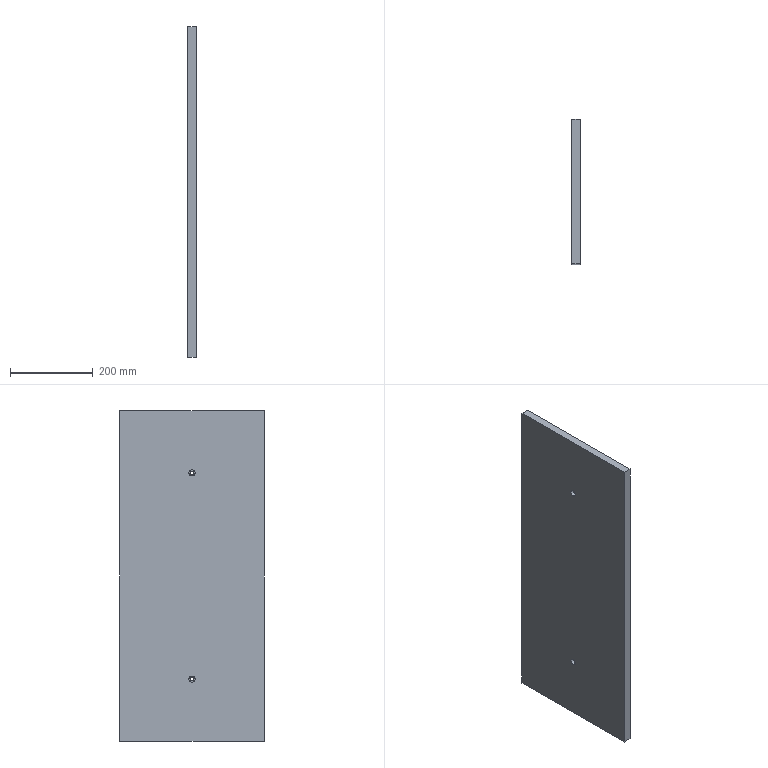Component | SolidWorks | ST60-10-1 | 1 solid | 16 faces | box 20 x 350 x 800 mm | volume 5595713 mm3 | cylinder 8 | plane 8 | commonest cylinder face diameters 15 x4 8 x4
build123d program:
from build123d import *

# Parameters (mm, degrees)
SKETCH1_W                                          = 800
SKETCH1_H                                          = 350
BOSS_EXTRUDE1_DEPTH                                = 20
HOLE_SIZE_ACCORDING_TO_TYPE_1_OF_HEXAG_D           = 8
HOLE_SIZE_ACCORDING_TO_TYPE_1_OF_HEXAG_CBORE_D     = 15
HOLE_SIZE_ACCORDING_TO_TYPE_1_OF_HEXAG_CBORE_DEPTH = 9


with BuildPart() as part:
    # Sketch1 → Boss-Extrude1 (new body)
    with BuildSketch(Plane.XY):
        with Locations((-1124.489, 541.975)):
            Rectangle(SKETCH1_W, SKETCH1_H)
    extrude(amount=BOSS_EXTRUDE1_DEPTH)

    # Hole Size _According to_ Type 1 of Hexag (through all)
    with Locations(Plane.XY.offset(20)):
        with Locations((-1374.489, 541.975), (-874.489, 541.975)):
            CounterBoreHole(HOLE_SIZE_ACCORDING_TO_TYPE_1_OF_HEXAG_D / 2, HOLE_SIZE_ACCORDING_TO_TYPE_1_OF_HEXAG_CBORE_D / 2, HOLE_SIZE_ACCORDING_TO_TYPE_1_OF_HEXAG_CBORE_DEPTH)


solid = part.part

# Placed as in the assembly
solid = solid.moved(Location((151.993, 68.479, -776.911), (0, -90, 0)))
STEP:
#1=COLOUR_RGB('',0.7922,0.8196,0.9333);
#2=FILL_AREA_STYLE_COLOUR('',#1);
#3=FILL_AREA_STYLE('',(#2));
#4=SURFACE_STYLE_FILL_AREA(#3);
#5=SURFACE_SIDE_STYLE('',(#4));
#6=SURFACE_STYLE_USAGE(.BOTH.,#5);
#7=PRESENTATION_STYLE_ASSIGNMENT((#6));
#8=CARTESIAN_POINT('',(5.551,24.034,-84.996));
#9=VERTEX_POINT('',#8);
#10=CARTESIAN_POINT('',(5.551,24.034,-84.406));
#11=VERTEX_POINT('',#10);
#12=CARTESIAN_POINT('',(5.551,24.034,-84.701));
#13=DIRECTION('',(-1.,-0.,0.));
#14=DIRECTION('',(0.,0.,1.));
#15=AXIS2_PLACEMENT_3D('',#12,#13,#14);
#16=CIRCLE('',#15,0.2953);
#17=EDGE_CURVE('',#9,#11,#16,.T.);
#18=ORIENTED_EDGE('',*,*,#17,.F.);
#19=CARTESIAN_POINT('',(5.197,24.034,-84.996));
#20=VERTEX_POINT('',#19);
#21=CARTESIAN_POINT('',(5.197,24.034,-84.996));
#22=DIRECTION('',(-1.,-0.,0.));
#23=VECTOR('',#22,39.37);
#24=LINE('',#21,#23);
#25=EDGE_CURVE('',#9,#20,#24,.T.);
#26=ORIENTED_EDGE('',*,*,#25,.T.);
#27=CARTESIAN_POINT('',(5.197,24.034,-84.406));
#28=VERTEX_POINT('',#27);
#29=CARTESIAN_POINT('',(5.197,24.034,-84.701));
#30=DIRECTION('',(-1.,-0.,0.));
#31=DIRECTION('',(0.,0.,1.));
#32=AXIS2_PLACEMENT_3D('',#29,#30,#31);
#33=CIRCLE('',#32,0.2953);
#34=EDGE_CURVE('',#20,#28,#33,.T.);
#35=ORIENTED_EDGE('',*,*,#34,.T.);
#36=CARTESIAN_POINT('',(5.197,24.034,-84.406));
#37=DIRECTION('',(-1.,-0.,0.));
#38=VECTOR('',#37,39.37);
#39=LINE('',#36,#38);
#40=EDGE_CURVE('',#11,#28,#39,.T.);
#41=ORIENTED_EDGE('',*,*,#40,.F.);
#42=EDGE_LOOP('',(#18,#26,#35,#41));
#43=FACE_OUTER_BOUND('',#42,.T.);
#44=CARTESIAN_POINT('',(5.197,24.034,-84.701));
#45=DIRECTION('',(-1.,-0.,0.));
#46=DIRECTION('',(0.,0.,1.));
#47=AXIS2_PLACEMENT_3D('',#44,#45,#46);
#48=CYLINDRICAL_SURFACE('',#47,0.2953);
#49=ADVANCED_FACE('',(#43),#48,.F.);
#50=CARTESIAN_POINT('',(5.984,24.034,-84.858));
#51=VERTEX_POINT('',#50);
#52=CARTESIAN_POINT('',(5.984,24.034,-84.543));
#53=VERTEX_POINT('',#52);
#54=CARTESIAN_POINT('',(5.984,24.034,-84.701));
#55=DIRECTION('',(-1.,-0.,0.));
#56=DIRECTION('',(0.,0.,1.));
#57=AXIS2_PLACEMENT_3D('',#54,#55,#56);
#58=CIRCLE('',#57,0.1575);
#59=EDGE_CURVE('',#51,#53,#58,.T.);
#60=ORIENTED_EDGE('',*,*,#59,.F.);
#61=CARTESIAN_POINT('',(5.551,24.034,-84.858));
#62=VERTEX_POINT('',#61);
#63=CARTESIAN_POINT('',(5.197,24.034,-84.858));
#64=DIRECTION('',(-1.,-0.,0.));
#65=VECTOR('',#64,39.37);
#66=LINE('',#63,#65);
#67=EDGE_CURVE('',#51,#62,#66,.T.);
#68=ORIENTED_EDGE('',*,*,#67,.T.);
#69=CARTESIAN_POINT('',(5.551,24.034,-84.543));
#70=VERTEX_POINT('',#69);
#71=CARTESIAN_POINT('',(5.551,24.034,-84.701));
#72=DIRECTION('',(-1.,-0.,0.));
#73=DIRECTION('',(0.,0.,1.));
#74=AXIS2_PLACEMENT_3D('',#71,#72,#73);
#75=CIRCLE('',#74,0.1575);
#76=EDGE_CURVE('',#62,#70,#75,.T.);
#77=ORIENTED_EDGE('',*,*,#76,.T.);
#78=CARTESIAN_POINT('',(5.197,24.034,-84.543));
#79=DIRECTION('',(-1.,-0.,0.));
#80=VECTOR('',#79,39.37);
#81=LINE('',#78,#80);
#82=EDGE_CURVE('',#53,#70,#81,.T.);
#83=ORIENTED_EDGE('',*,*,#82,.F.);
#84=EDGE_LOOP('',(#60,#68,#77,#83));
#85=FACE_OUTER_BOUND('',#84,.T.);
#86=CARTESIAN_POINT('',(5.197,24.034,-84.701));
#87=DIRECTION('',(-1.,-0.,0.));
#88=DIRECTION('',(0.,0.,1.));
#89=AXIS2_PLACEMENT_3D('',#86,#87,#88);
#90=CYLINDRICAL_SURFACE('',#89,0.1575);
#91=ADVANCED_FACE('',(#85),#90,.F.);
#92=CARTESIAN_POINT('',(5.551,24.034,-65.311));
#93=VERTEX_POINT('',#92);
#94=CARTESIAN_POINT('',(5.551,24.034,-64.72));
#95=VERTEX_POINT('',#94);
#96=CARTESIAN_POINT('',(5.551,24.034,-65.016));
#97=DIRECTION('',(-1.,-0.,0.));
#98=DIRECTION('',(0.,0.,1.));
#99=AXIS2_PLACEMENT_3D('',#96,#97,#98);
#100=CIRCLE('',#99,0.2953);
#101=EDGE_CURVE('',#93,#95,#100,.T.);
#102=ORIENTED_EDGE('',*,*,#101,.F.);
#103=CARTESIAN_POINT('',(5.197,24.034,-65.311));
#104=VERTEX_POINT('',#103);
#105=CARTESIAN_POINT('',(5.197,24.034,-65.311));
#106=DIRECTION('',(-1.,-0.,0.));
#107=VECTOR('',#106,39.37);
#108=LINE('',#105,#107);
#109=EDGE_CURVE('',#93,#104,#108,.T.);
#110=ORIENTED_EDGE('',*,*,#109,.T.);
#111=CARTESIAN_POINT('',(5.197,24.034,-64.72));
#112=VERTEX_POINT('',#111);
#113=CARTESIAN_POINT('',(5.197,24.034,-65.016));
#114=DIRECTION('',(-1.,-0.,0.));
#115=DIRECTION('',(0.,0.,1.));
#116=AXIS2_PLACEMENT_3D('',#113,#114,#115);
#117=CIRCLE('',#116,0.2953);
#118=EDGE_CURVE('',#104,#112,#117,.T.);
#119=ORIENTED_EDGE('',*,*,#118,.T.);
#120=CARTESIAN_POINT('',(5.197,24.034,-64.72));
#121=DIRECTION('',(-1.,-0.,0.));
#122=VECTOR('',#121,39.37);
#123=LINE('',#120,#122);
#124=EDGE_CURVE('',#95,#112,#123,.T.);
#125=ORIENTED_EDGE('',*,*,#124,.F.);
#126=EDGE_LOOP('',(#102,#110,#119,#125));
#127=FACE_OUTER_BOUND('',#126,.T.);
#128=CARTESIAN_POINT('',(5.197,24.034,-65.016));
#129=DIRECTION('',(-1.,-0.,0.));
#130=DIRECTION('',(0.,0.,1.));
#131=AXIS2_PLACEMENT_3D('',#128,#129,#130);
#132=CYLINDRICAL_SURFACE('',#131,0.2953);
#133=ADVANCED_FACE('',(#127),#132,.F.);
#134=CARTESIAN_POINT('',(5.984,24.034,-65.173));
#135=VERTEX_POINT('',#134);
#136=CARTESIAN_POINT('',(5.984,24.034,-64.858));
#137=VERTEX_POINT('',#136);
#138=CARTESIAN_POINT('',(5.984,24.034,-65.016));
#139=DIRECTION('',(-1.,-0.,0.));
#140=DIRECTION('',(0.,0.,1.));
#141=AXIS2_PLACEMENT_3D('',#138,#139,#140);
#142=CIRCLE('',#141,0.1575);
#143=EDGE_CURVE('',#135,#137,#142,.T.);
#144=ORIENTED_EDGE('',*,*,#143,.F.);
#145=CARTESIAN_POINT('',(5.551,24.034,-65.173));
#146=VERTEX_POINT('',#145);
#147=CARTESIAN_POINT('',(5.197,24.034,-65.173));
#148=DIRECTION('',(-1.,-0.,0.));
#149=VECTOR('',#148,39.37);
#150=LINE('',#147,#149);
#151=EDGE_CURVE('',#135,#146,#150,.T.);
#152=ORIENTED_EDGE('',*,*,#151,.T.);
#153=CARTESIAN_POINT('',(5.551,24.034,-64.858));
#154=VERTEX_POINT('',#153);
#155=CARTESIAN_POINT('',(5.551,24.034,-65.016));
#156=DIRECTION('',(-1.,-0.,0.));
#157=DIRECTION('',(0.,0.,1.));
#158=AXIS2_PLACEMENT_3D('',#155,#156,#157);
#159=CIRCLE('',#158,0.1575);
#160=EDGE_CURVE('',#146,#154,#159,.T.);
#161=ORIENTED_EDGE('',*,*,#160,.T.);
#162=CARTESIAN_POINT('',(5.197,24.034,-64.858));
#163=DIRECTION('',(-1.,-0.,0.));
#164=VECTOR('',#163,39.37);
#165=LINE('',#162,#164);
#166=EDGE_CURVE('',#137,#154,#165,.T.);
#167=ORIENTED_EDGE('',*,*,#166,.F.);
#168=EDGE_LOOP('',(#144,#152,#161,#167));
#169=FACE_OUTER_BOUND('',#168,.T.);
#170=CARTESIAN_POINT('',(5.197,24.034,-65.016));
#171=DIRECTION('',(-1.,-0.,0.));
#172=DIRECTION('',(0.,0.,1.));
#173=AXIS2_PLACEMENT_3D('',#170,#171,#172);
#174=CYLINDRICAL_SURFACE('',#173,0.1575);
#175=ADVANCED_FACE('',(#169),#174,.F.);
#176=CARTESIAN_POINT('',(5.984,30.923,-90.606));
#177=VERTEX_POINT('',#176);
#178=CARTESIAN_POINT('',(5.984,17.144,-90.606));
#179=VERTEX_POINT('',#178);
#180=CARTESIAN_POINT('',(5.984,30.923,-90.606));
#181=DIRECTION('',(0.,-1.,0.));
#182=VECTOR('',#181,39.37);
#183=LINE('',#180,#182);
#184=EDGE_CURVE('',#177,#179,#183,.T.);
#185=ORIENTED_EDGE('',*,*,#184,.T.);
#186=CARTESIAN_POINT('',(5.197,17.144,-90.606));
#187=VERTEX_POINT('',#186);
#188=CARTESIAN_POINT('',(5.197,17.144,-90.606));
#189=DIRECTION('',(1.,0.,-0.));
#190=VECTOR('',#189,39.37);
#191=LINE('',#188,#190);
#192=EDGE_CURVE('',#187,#179,#191,.T.);
#193=ORIENTED_EDGE('',*,*,#192,.F.);
#194=CARTESIAN_POINT('',(5.197,30.923,-90.606));
#195=VERTEX_POINT('',#194);
#196=CARTESIAN_POINT('',(5.197,30.923,-90.606));
#197=DIRECTION('',(0.,-1.,0.));
#198=VECTOR('',#197,39.37);
#199=LINE('',#196,#198);
#200=EDGE_CURVE('',#195,#187,#199,.T.);
#201=ORIENTED_EDGE('',*,*,#200,.F.);
#202=CARTESIAN_POINT('',(5.197,30.923,-90.606));
#203=DIRECTION('',(1.,0.,-0.));
#204=VECTOR('',#203,39.37);
#205=LINE('',#202,#204);
#206=EDGE_CURVE('',#195,#177,#205,.T.);
#207=ORIENTED_EDGE('',*,*,#206,.T.);
#208=EDGE_LOOP('',(#185,#193,#201,#207));
#209=FACE_OUTER_BOUND('',#208,.T.);
#210=CARTESIAN_POINT('',(5.197,30.923,-90.606));
#211=DIRECTION('',(0.,0.,1.));
#212=DIRECTION('',(-0.,1.,-0.));
#213=AXIS2_PLACEMENT_3D('',#210,#211,#212);
#214=PLANE('',#213);
#215=ADVANCED_FACE('',(#209),#214,.F.);
#216=CARTESIAN_POINT('',(5.984,17.144,-59.11));
#217=VERTEX_POINT('',#216);
#218=CARTESIAN_POINT('',(5.984,17.144,-90.606));
#219=DIRECTION('',(0.,-0.,1.));
#220=VECTOR('',#219,39.37);
#221=LINE('',#218,#220);
#222=EDGE_CURVE('',#179,#217,#221,.T.);
#223=ORIENTED_EDGE('',*,*,#222,.T.);
#224=CARTESIAN_POINT('',(5.197,17.144,-59.11));
#225=VERTEX_POINT('',#224);
#226=CARTESIAN_POINT('',(5.197,17.144,-59.11));
#227=DIRECTION('',(1.,0.,-0.));
#228=VECTOR('',#227,39.37);
#229=LINE('',#226,#228);
#230=EDGE_CURVE('',#225,#217,#229,.T.);
#231=ORIENTED_EDGE('',*,*,#230,.F.);
#232=CARTESIAN_POINT('',(5.197,17.144,-90.606));
#233=DIRECTION('',(0.,-0.,1.));
#234=VECTOR('',#233,39.37);
#235=LINE('',#232,#234);
#236=EDGE_CURVE('',#187,#225,#235,.T.);
#237=ORIENTED_EDGE('',*,*,#236,.F.);
#238=ORIENTED_EDGE('',*,*,#192,.T.);
#239=EDGE_LOOP('',(#223,#231,#237,#238));
#240=FACE_OUTER_BOUND('',#239,.T.);
#241=CARTESIAN_POINT('',(5.197,17.144,-90.606));
#242=DIRECTION('',(-0.,1.,0.));
#243=DIRECTION('',(-1.,-0.,0.));
#244=AXIS2_PLACEMENT_3D('',#241,#242,#243);
#245=PLANE('',#244);
#246=ADVANCED_FACE('',(#240),#245,.F.);
#247=CARTESIAN_POINT('',(5.984,30.923,-59.11));
#248=VERTEX_POINT('',#247);
#249=CARTESIAN_POINT('',(5.984,30.923,-59.11));
#250=DIRECTION('',(-0.,1.,0.));
#251=VECTOR('',#250,39.37);
#252=LINE('',#249,#251);
#253=EDGE_CURVE('',#217,#248,#252,.T.);
#254=ORIENTED_EDGE('',*,*,#253,.T.);
#255=CARTESIAN_POINT('',(5.197,30.923,-59.11));
#256=VERTEX_POINT('',#255);
#257=CARTESIAN_POINT('',(5.197,30.923,-59.11));
#258=DIRECTION('',(1.,0.,-0.));
#259=VECTOR('',#258,39.37);
#260=LINE('',#257,#259);
#261=EDGE_CURVE('',#256,#248,#260,.T.);
#262=ORIENTED_EDGE('',*,*,#261,.F.);
#263=CARTESIAN_POINT('',(5.197,30.923,-59.11));
#264=DIRECTION('',(-0.,1.,0.));
#265=VECTOR('',#264,39.37);
#266=LINE('',#263,#265);
#267=EDGE_CURVE('',#225,#256,#266,.T.);
#268=ORIENTED_EDGE('',*,*,#267,.F.);
#269=ORIENTED_EDGE('',*,*,#230,.T.);
#270=EDGE_LOOP('',(#254,#262,#268,#269));
#271=FACE_OUTER_BOUND('',#270,.T.);
#272=CARTESIAN_POINT('',(5.197,30.923,-59.11));
#273=DIRECTION('',(-0.,0.,-1.));
#274=DIRECTION('',(-1.,-0.,0.));
#275=AXIS2_PLACEMENT_3D('',#272,#273,#274);
#276=PLANE('',#275);
#277=ADVANCED_FACE('',(#271),#276,.F.);
#278=CARTESIAN_POINT('',(5.984,30.923,-90.606));
#279=DIRECTION('',(-0.,0.,-1.));
#280=VECTOR('',#279,39.37);
#281=LINE('',#278,#280);
#282=EDGE_CURVE('',#248,#177,#281,.T.);
#283=ORIENTED_EDGE('',*,*,#282,.T.);
#284=ORIENTED_EDGE('',*,*,#206,.F.);
#285=CARTESIAN_POINT('',(5.197,30.923,-90.606));
#286=DIRECTION('',(-0.,0.,-1.));
#287=VECTOR('',#286,39.37);
#288=LINE('',#285,#287);
#289=EDGE_CURVE('',#256,#195,#288,.T.);
#290=ORIENTED_EDGE('',*,*,#289,.F.);
#291=ORIENTED_EDGE('',*,*,#261,.T.);
#292=EDGE_LOOP('',(#283,#284,#290,#291));
#293=FACE_OUTER_BOUND('',#292,.T.);
#294=CARTESIAN_POINT('',(5.197,30.923,-90.606));
#295=DIRECTION('',(0.,-1.,-0.));
#296=DIRECTION('',(1.,0.,-0.));
#297=AXIS2_PLACEMENT_3D('',#294,#295,#296);
#298=PLANE('',#297);
#299=ADVANCED_FACE('',(#293),#298,.F.);
#300=CARTESIAN_POINT('',(5.197,24.034,-84.701));
#301=DIRECTION('',(-1.,-0.,0.));
#302=DIRECTION('',(0.,0.,1.));
#303=AXIS2_PLACEMENT_3D('',#300,#301,#302);
#304=CIRCLE('',#303,0.2953);
#305=EDGE_CURVE('',#28,#20,#304,.T.);
#306=ORIENTED_EDGE('',*,*,#305,.F.);
#307=ORIENTED_EDGE('',*,*,#34,.F.);
#308=EDGE_LOOP('',(#306,#307));
#309=FACE_BOUND('',#308,.T.);
#310=CARTESIAN_POINT('',(5.197,24.034,-65.016));
#311=DIRECTION('',(-1.,-0.,0.));
#312=DIRECTION('',(0.,0.,1.));
#313=AXIS2_PLACEMENT_3D('',#310,#311,#312);
#314=CIRCLE('',#313,0.2953);
#315=EDGE_CURVE('',#112,#104,#314,.T.);
#316=ORIENTED_EDGE('',*,*,#315,.F.);
#317=ORIENTED_EDGE('',*,*,#118,.F.);
#318=EDGE_LOOP('',(#316,#317));
#319=FACE_BOUND('',#318,.T.);
#320=ORIENTED_EDGE('',*,*,#200,.T.);
#321=ORIENTED_EDGE('',*,*,#236,.T.);
#322=ORIENTED_EDGE('',*,*,#267,.T.);
#323=ORIENTED_EDGE('',*,*,#289,.T.);
#324=EDGE_LOOP('',(#320,#321,#322,#323));
#325=FACE_OUTER_BOUND('',#324,.T.);
#326=CARTESIAN_POINT('',(5.197,2.696,-30.587));
#327=DIRECTION('',(-1.,-0.,0.));
#328=DIRECTION('',(0.,-0.,1.));
#329=AXIS2_PLACEMENT_3D('',#326,#327,#328);
#330=PLANE('',#329);
#331=ADVANCED_FACE('',(#309,#319,#325),#330,.T.);
#332=CARTESIAN_POINT('',(5.984,24.034,-84.701));
#333=DIRECTION('',(-1.,-0.,0.));
#334=DIRECTION('',(0.,0.,1.));
#335=AXIS2_PLACEMENT_3D('',#332,#333,#334);
#336=CIRCLE('',#335,0.1575);
#337=EDGE_CURVE('',#53,#51,#336,.T.);
#338=ORIENTED_EDGE('',*,*,#337,.T.);
#339=ORIENTED_EDGE('',*,*,#59,.T.);
#340=EDGE_LOOP('',(#338,#339));
#341=FACE_BOUND('',#340,.T.);
#342=CARTESIAN_POINT('',(5.984,24.034,-65.016));
#343=DIRECTION('',(-1.,-0.,0.));
#344=DIRECTION('',(0.,0.,1.));
#345=AXIS2_PLACEMENT_3D('',#342,#343,#344);
#346=CIRCLE('',#345,0.1575);
#347=EDGE_CURVE('',#137,#135,#346,.T.);
#348=ORIENTED_EDGE('',*,*,#347,.T.);
#349=ORIENTED_EDGE('',*,*,#143,.T.);
#350=EDGE_LOOP('',(#348,#349));
#351=FACE_BOUND('',#350,.T.);
#352=ORIENTED_EDGE('',*,*,#184,.F.);
#353=ORIENTED_EDGE('',*,*,#282,.F.);
#354=ORIENTED_EDGE('',*,*,#253,.F.);
#355=ORIENTED_EDGE('',*,*,#222,.F.);
#356=EDGE_LOOP('',(#352,#353,#354,#355));
#357=FACE_OUTER_BOUND('',#356,.T.);
#358=CARTESIAN_POINT('',(5.984,2.696,-30.587));
#359=DIRECTION('',(-1.,-0.,0.));
#360=DIRECTION('',(0.,-0.,1.));
#361=AXIS2_PLACEMENT_3D('',#358,#359,#360);
#362=PLANE('',#361);
#363=ADVANCED_FACE('',(#341,#351,#357),#362,.F.);
#364=ORIENTED_EDGE('',*,*,#151,.F.);
#365=ORIENTED_EDGE('',*,*,#347,.F.);
#366=ORIENTED_EDGE('',*,*,#166,.T.);
#367=CARTESIAN_POINT('',(5.551,24.034,-65.016));
#368=DIRECTION('',(-1.,-0.,0.));
#369=DIRECTION('',(0.,0.,1.));
#370=AXIS2_PLACEMENT_3D('',#367,#368,#369);
#371=CIRCLE('',#370,0.1575);
#372=EDGE_CURVE('',#154,#146,#371,.T.);
#373=ORIENTED_EDGE('',*,*,#372,.T.);
#374=EDGE_LOOP('',(#364,#365,#366,#373));
#375=FACE_OUTER_BOUND('',#374,.T.);
#376=CARTESIAN_POINT('',(5.197,24.034,-65.016));
#377=DIRECTION('',(-1.,-0.,0.));
#378=DIRECTION('',(0.,0.,1.));
#379=AXIS2_PLACEMENT_3D('',#376,#377,#378);
#380=CYLINDRICAL_SURFACE('',#379,0.1575);
#381=ADVANCED_FACE('',(#375),#380,.F.);
#382=ORIENTED_EDGE('',*,*,#372,.F.);
#383=ORIENTED_EDGE('',*,*,#160,.F.);
#384=EDGE_LOOP('',(#382,#383));
#385=FACE_BOUND('',#384,.T.);
#386=CARTESIAN_POINT('',(5.551,24.034,-65.016));
#387=DIRECTION('',(-1.,-0.,0.));
#388=DIRECTION('',(0.,0.,1.));
#389=AXIS2_PLACEMENT_3D('',#386,#387,#388);
#390=CIRCLE('',#389,0.2953);
#391=EDGE_CURVE('',#95,#93,#390,.T.);
#392=ORIENTED_EDGE('',*,*,#391,.T.);
#393=ORIENTED_EDGE('',*,*,#101,.T.);
#394=EDGE_LOOP('',(#392,#393));
#395=FACE_OUTER_BOUND('',#394,.T.);
#396=CARTESIAN_POINT('',(5.551,24.034,-64.858));
#397=DIRECTION('',(1.,0.,-0.));
#398=DIRECTION('',(-0.,0.,-1.));
#399=AXIS2_PLACEMENT_3D('',#396,#397,#398);
#400=PLANE('',#399);
#401=ADVANCED_FACE('',(#385,#395),#400,.F.);
#402=ORIENTED_EDGE('',*,*,#109,.F.);
#403=ORIENTED_EDGE('',*,*,#391,.F.);
#404=ORIENTED_EDGE('',*,*,#124,.T.);
#405=ORIENTED_EDGE('',*,*,#315,.T.);
#406=EDGE_LOOP('',(#402,#403,#404,#405));
#407=FACE_OUTER_BOUND('',#406,.T.);
#408=CARTESIAN_POINT('',(5.197,24.034,-65.016));
#409=DIRECTION('',(-1.,-0.,0.));
#410=DIRECTION('',(0.,0.,1.));
#411=AXIS2_PLACEMENT_3D('',#408,#409,#410);
#412=CYLINDRICAL_SURFACE('',#411,0.2953);
#413=ADVANCED_FACE('',(#407),#412,.F.);
#414=ORIENTED_EDGE('',*,*,#67,.F.);
#415=ORIENTED_EDGE('',*,*,#337,.F.);
#416=ORIENTED_EDGE('',*,*,#82,.T.);
#417=CARTESIAN_POINT('',(5.551,24.034,-84.701));
#418=DIRECTION('',(-1.,-0.,0.));
#419=DIRECTION('',(0.,0.,1.));
#420=AXIS2_PLACEMENT_3D('',#417,#418,#419);
#421=CIRCLE('',#420,0.1575);
#422=EDGE_CURVE('',#70,#62,#421,.T.);
#423=ORIENTED_EDGE('',*,*,#422,.T.);
#424=EDGE_LOOP('',(#414,#415,#416,#423));
#425=FACE_OUTER_BOUND('',#424,.T.);
#426=CARTESIAN_POINT('',(5.197,24.034,-84.701));
#427=DIRECTION('',(-1.,-0.,0.));
#428=DIRECTION('',(0.,0.,1.));
#429=AXIS2_PLACEMENT_3D('',#426,#427,#428);
#430=CYLINDRICAL_SURFACE('',#429,0.1575);
#431=ADVANCED_FACE('',(#425),#430,.F.);
#432=ORIENTED_EDGE('',*,*,#422,.F.);
#433=ORIENTED_EDGE('',*,*,#76,.F.);
#434=EDGE_LOOP('',(#432,#433));
#435=FACE_BOUND('',#434,.T.);
#436=CARTESIAN_POINT('',(5.551,24.034,-84.701));
#437=DIRECTION('',(-1.,-0.,0.));
#438=DIRECTION('',(0.,0.,1.));
#439=AXIS2_PLACEMENT_3D('',#436,#437,#438);
#440=CIRCLE('',#439,0.2953);
#441=EDGE_CURVE('',#11,#9,#440,.T.);
#442=ORIENTED_EDGE('',*,*,#441,.T.);
#443=ORIENTED_EDGE('',*,*,#17,.T.);
#444=EDGE_LOOP('',(#442,#443));
#445=FACE_OUTER_BOUND('',#444,.T.);
#446=CARTESIAN_POINT('',(5.551,24.034,-84.543));
#447=DIRECTION('',(1.,0.,-0.));
#448=DIRECTION('',(-0.,0.,-1.));
#449=AXIS2_PLACEMENT_3D('',#446,#447,#448);
#450=PLANE('',#449);
#451=ADVANCED_FACE('',(#435,#445),#450,.F.);
#452=ORIENTED_EDGE('',*,*,#25,.F.);
#453=ORIENTED_EDGE('',*,*,#441,.F.);
#454=ORIENTED_EDGE('',*,*,#40,.T.);
#455=ORIENTED_EDGE('',*,*,#305,.T.);
#456=EDGE_LOOP('',(#452,#453,#454,#455));
#457=FACE_OUTER_BOUND('',#456,.T.);
#458=CARTESIAN_POINT('',(5.197,24.034,-84.701));
#459=DIRECTION('',(-1.,-0.,0.));
#460=DIRECTION('',(0.,0.,1.));
#461=AXIS2_PLACEMENT_3D('',#458,#459,#460);
#462=CYLINDRICAL_SURFACE('',#461,0.2953);
#463=ADVANCED_FACE('',(#457),#462,.F.);
#464=CLOSED_SHELL('',(#49,#91,#133,#175,#215,#246,#277,#299,#331,#363,#381,#401,#413,#431,#451,#463));
#465=MANIFOLD_SOLID_BREP('',#464);
#466=STYLED_ITEM('',(#7),#465);
#467=(LENGTH_UNIT()NAMED_UNIT(*)SI_UNIT($,.METRE.));
#468=LENGTH_MEASURE_WITH_UNIT(LENGTH_MEASURE(0.0254),#467);
#469=DIMENSIONAL_EXPONENTS(1.,0.,0.,0.,0.,0.,0.);
#470=(CONVERSION_BASED_UNIT('',#468)LENGTH_UNIT()NAMED_UNIT(#469));
#471=UNCERTAINTY_MEASURE_WITH_UNIT(LENGTH_MEASURE(0.00001),#470,'','');
#472=(NAMED_UNIT(*)PLANE_ANGLE_UNIT()SI_UNIT($,.RADIAN.));
#473=(NAMED_UNIT(*)SI_UNIT($,.STERADIAN.)SOLID_ANGLE_UNIT());
#474=(GEOMETRIC_REPRESENTATION_CONTEXT(3)GLOBAL_UNCERTAINTY_ASSIGNED_CONTEXT((#471))GLOBAL_UNIT_ASSIGNED_CONTEXT((#470,#472,#473))REPRESENTATION_CONTEXT('',''));
#475=MECHANICAL_DESIGN_GEOMETRIC_PRESENTATION_REPRESENTATION('',(#466),#474);
#476=PRESENTATION_LAYER_ASSIGNMENT('','',(#466));
#477=CARTESIAN_POINT('',(0.,0.,0.));
#478=DIRECTION('',(0.,0.,1.));
#479=DIRECTION('',(1.,0.,0.));
#480=AXIS2_PLACEMENT_3D('',#477,#478,#479);
#481=(LENGTH_UNIT()NAMED_UNIT(*)SI_UNIT($,.METRE.));
#482=LENGTH_MEASURE_WITH_UNIT(LENGTH_MEASURE(0.0254),#481);
#483=DIMENSIONAL_EXPONENTS(1.,0.,0.,0.,0.,0.,0.);
#484=(CONVERSION_BASED_UNIT('',#482)LENGTH_UNIT()NAMED_UNIT(#483));
#485=UNCERTAINTY_MEASURE_WITH_UNIT(LENGTH_MEASURE(0.00001),#484,'','');
#486=(NAMED_UNIT(*)PLANE_ANGLE_UNIT()SI_UNIT($,.RADIAN.));
#487=(NAMED_UNIT(*)SI_UNIT($,.STERADIAN.)SOLID_ANGLE_UNIT());
#488=(GEOMETRIC_REPRESENTATION_CONTEXT(3)GLOBAL_UNCERTAINTY_ASSIGNED_CONTEXT((#485))GLOBAL_UNIT_ASSIGNED_CONTEXT((#484,#486,#487))REPRESENTATION_CONTEXT('',''));
#489=ADVANCED_BREP_SHAPE_REPRESENTATION('',(#465,#480),#488);